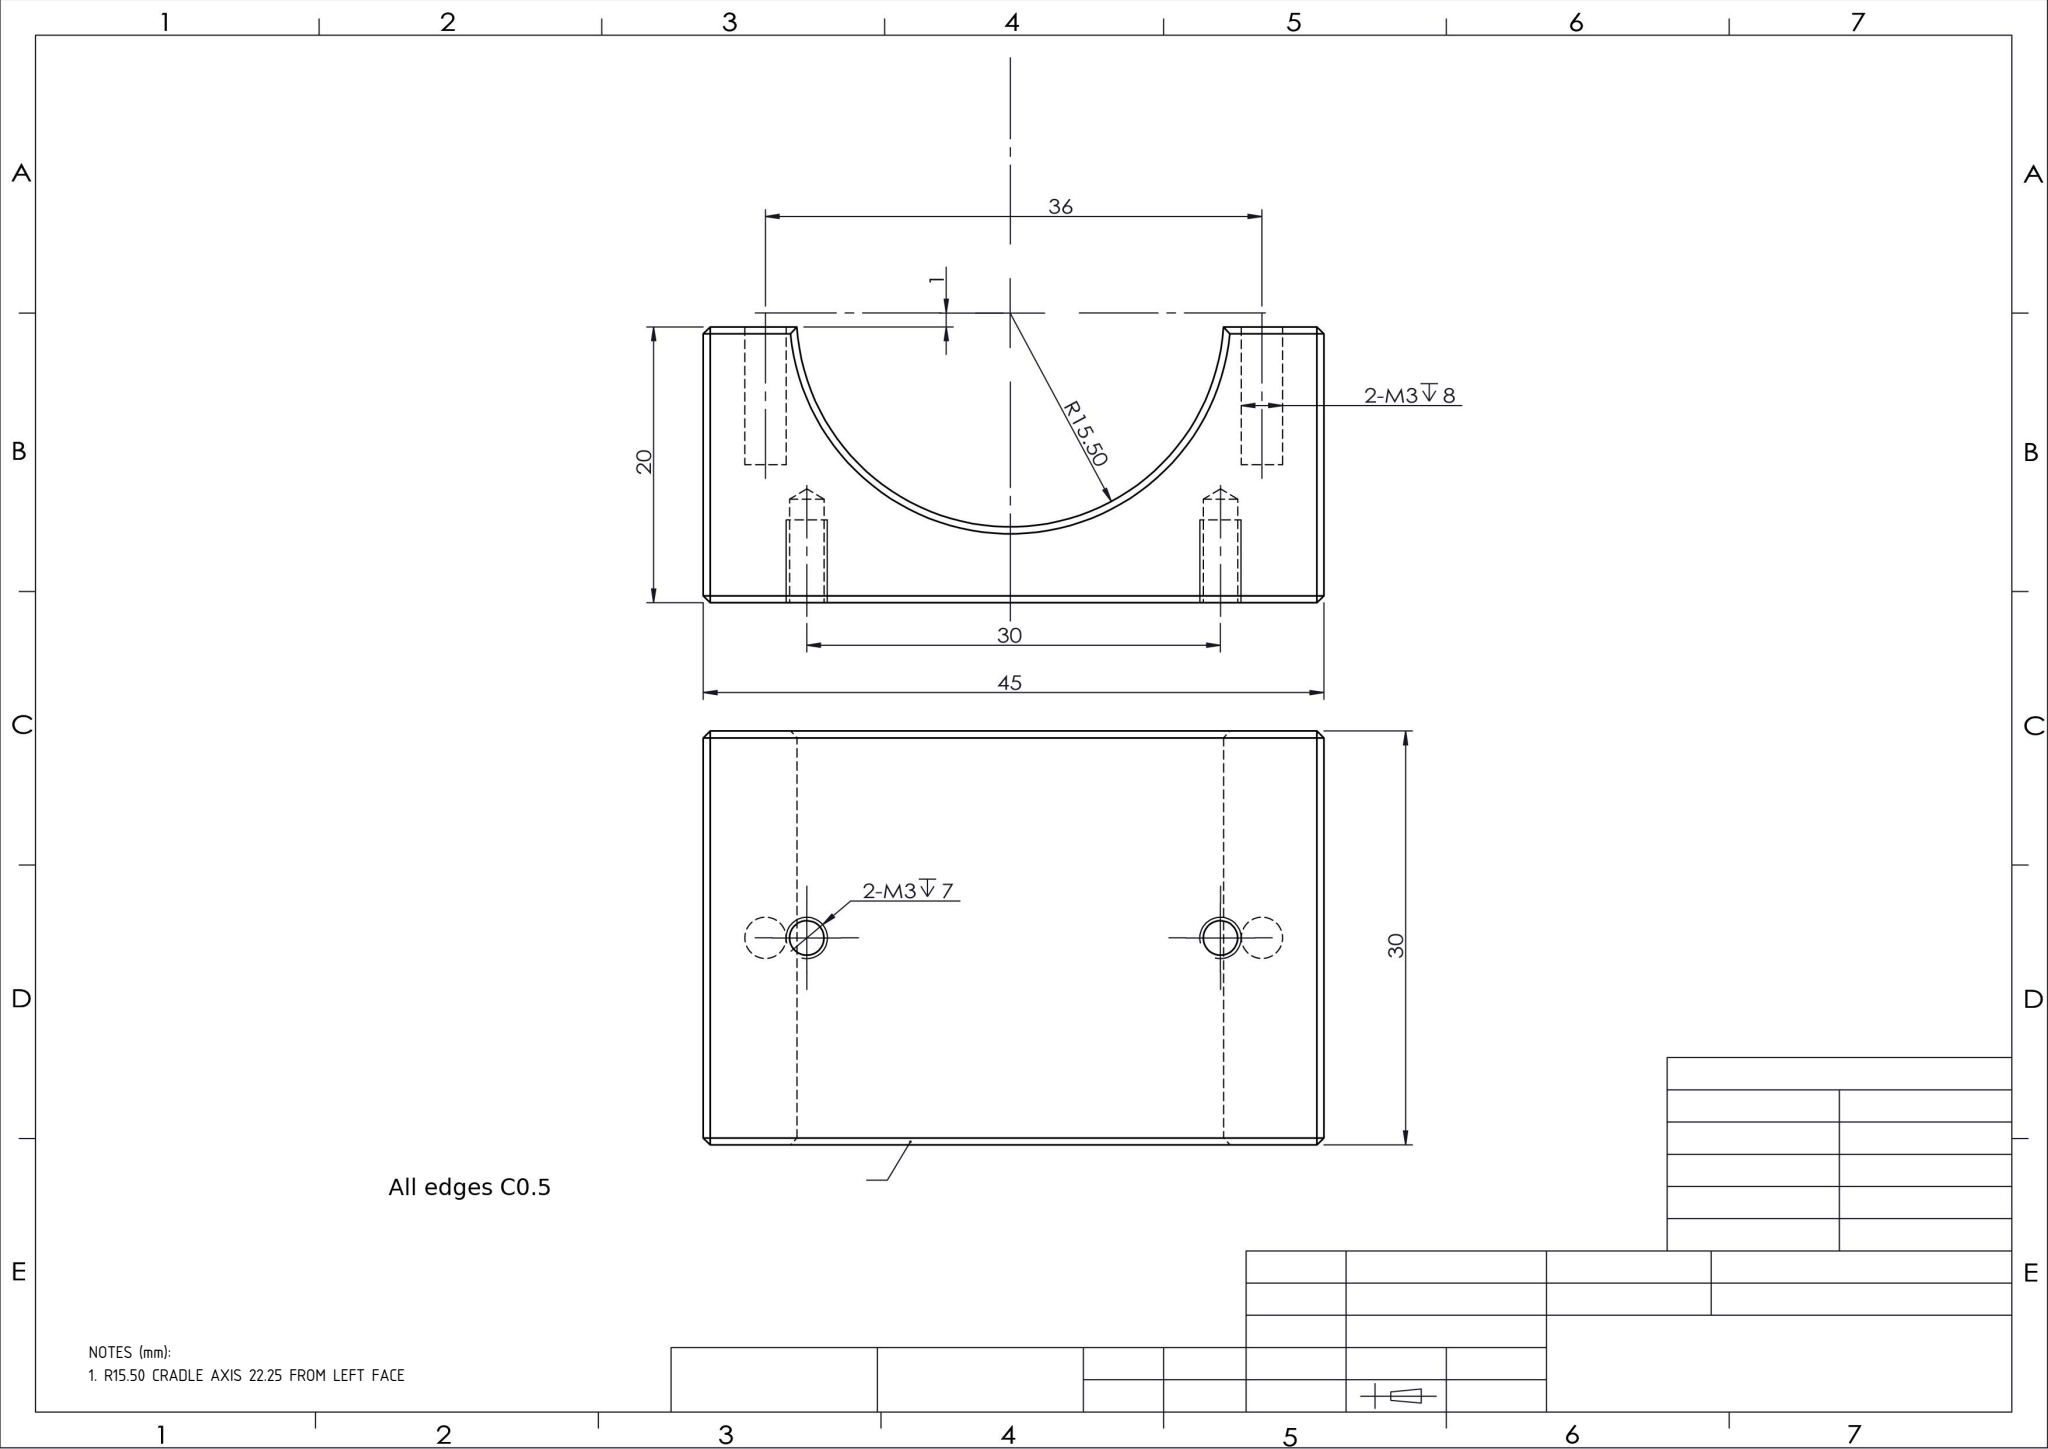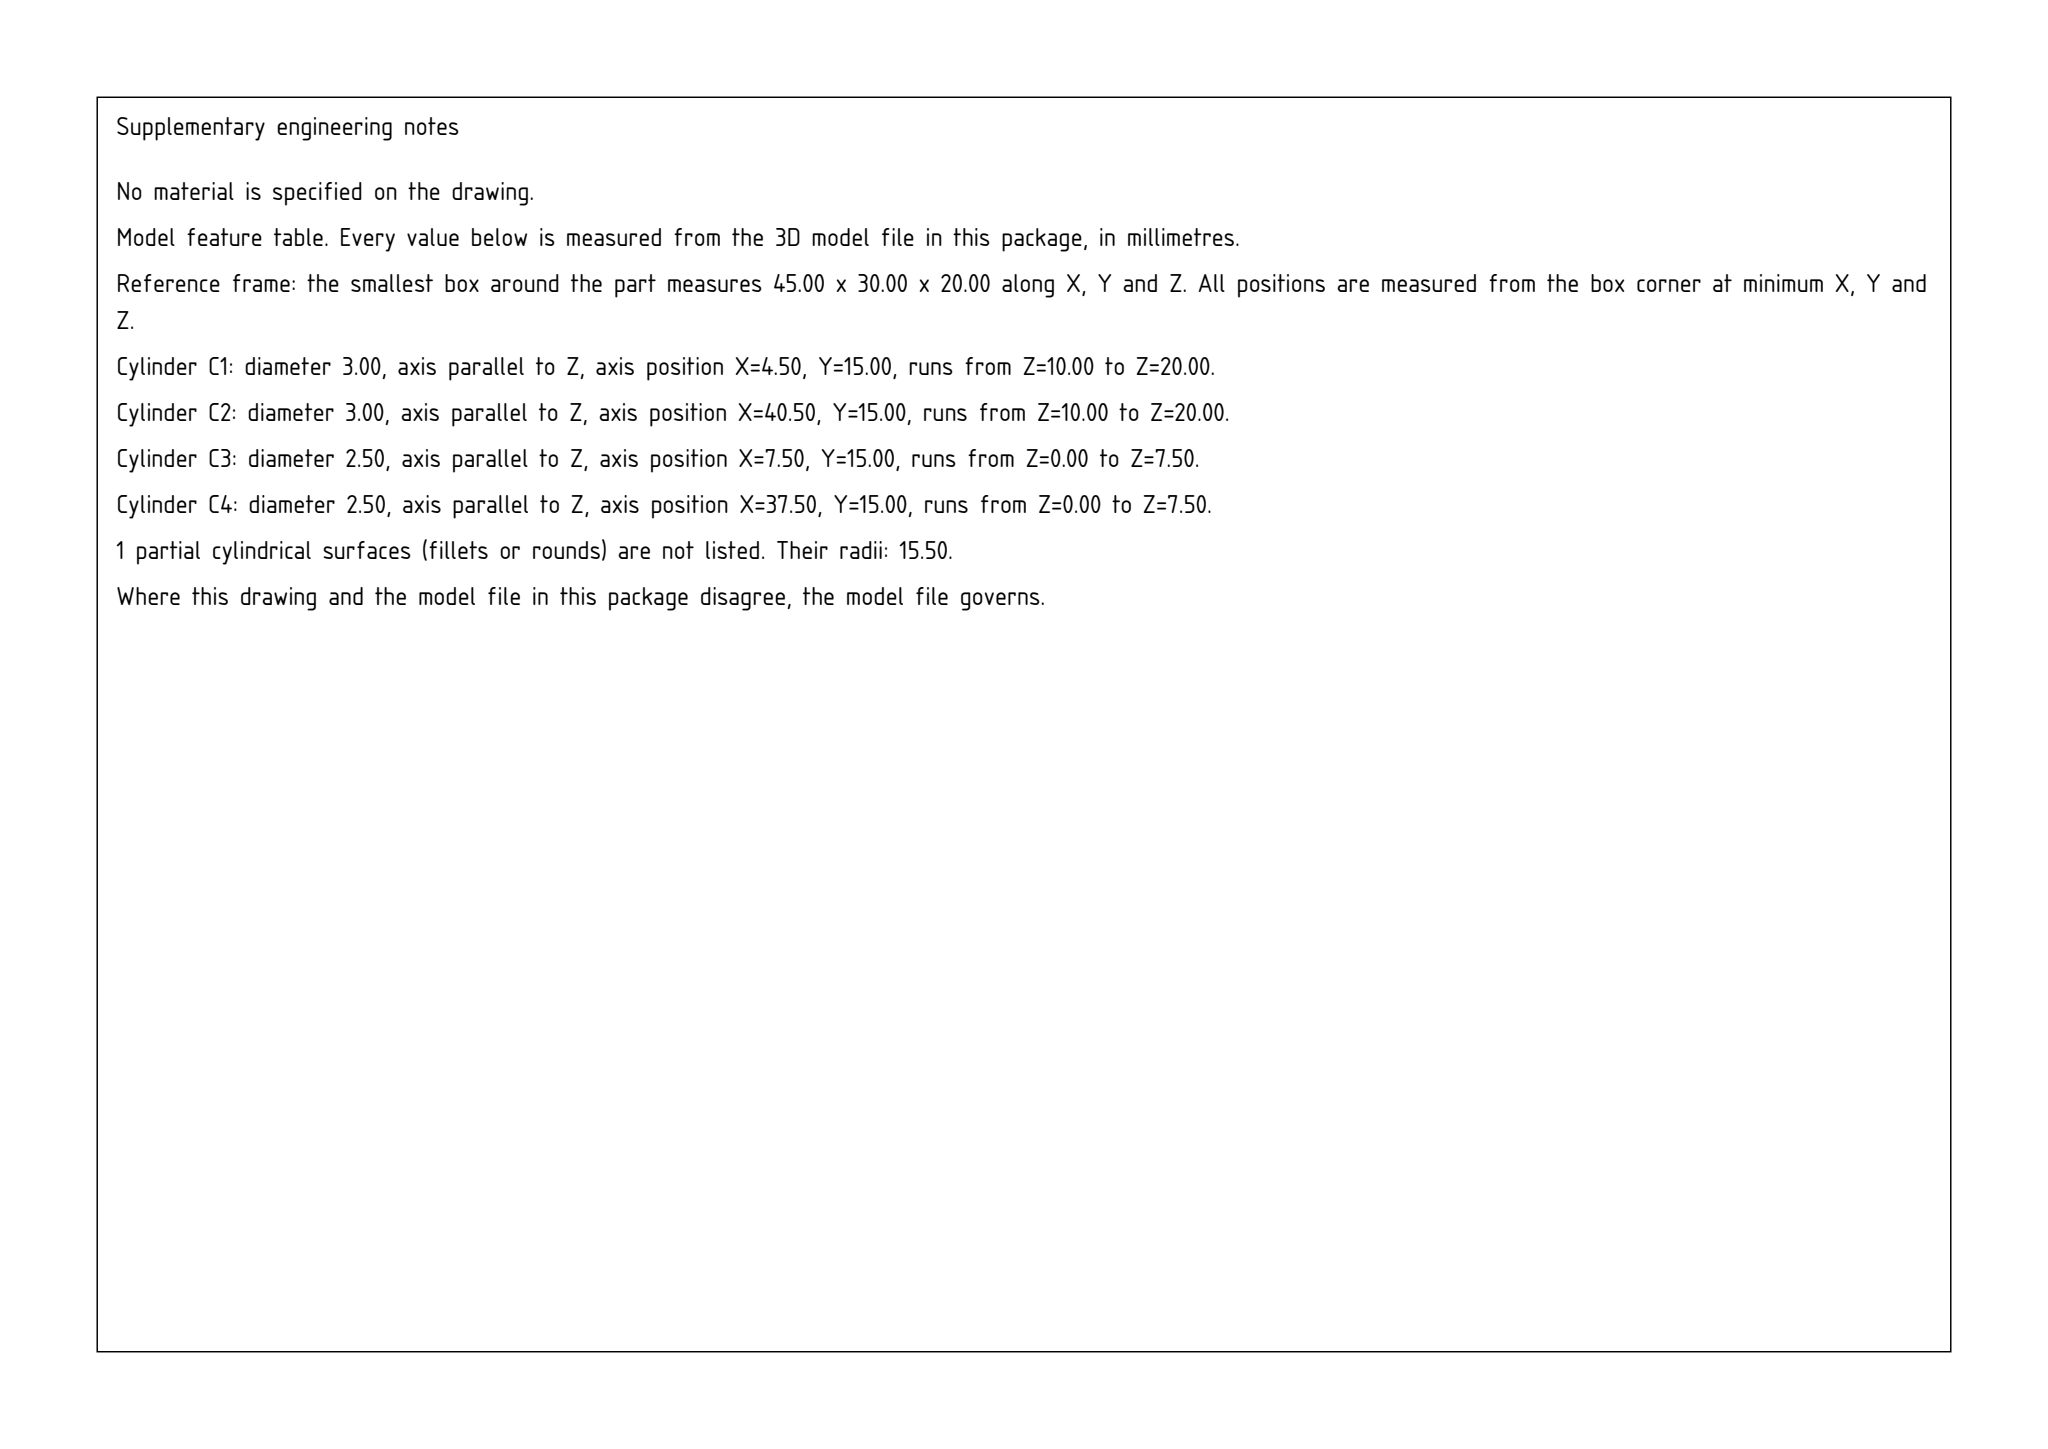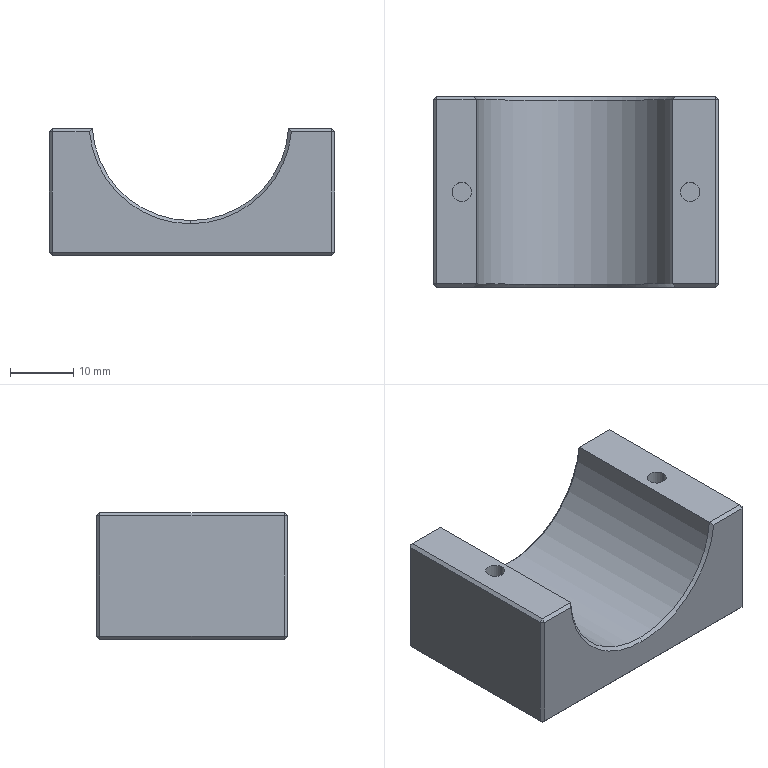Part | SolidWorks | mm | 1 solid | 47 faces | box 45 x 30 x 20 mm | volume 16340 mm3 | plane 31 | cylinder 9 | cone 7 | commonest cylinder face diameters 2.5 x4 3 x4 31 x1
Drawing notes:
R15.50 CRADLE AXIS 22.25 FROM LEFT FACE | from the solid: cylinder dia 31.0 axis y at x=22.25 (bbox x 0-45)
build123d program:
from build123d import *

# Parameters (mm, degrees)
SKETCH1_W             = 45
SKETCH1_H             = 30
BOSS_EXTRUDE1_DEPTH   = 20
SKETCH2_R             = 15.5
CUT_EXTRUDE1_DEPTH    = 58.663
SKETCH3_R             = 1.5
CUT_EXTRUDE2_DEPTH    = 10
M3_TAPPED_HOLE1_D     = 2.5
M3_TAPPED_HOLE1_DEPTH = 7.5
M3_TAPPED_HOLE1_TIP   = 0.7511
CHAMFER1_SIZE         = 0.5


with BuildPart() as part:
    # Sketch1 → Boss-Extrude1 (new body)
    with BuildSketch(Plane.XY):
        with Locations((22.5, 15)):
            Rectangle(SKETCH1_W, SKETCH1_H)
    extrude(amount=BOSS_EXTRUDE1_DEPTH)

    # Sketch2 → Cut-Extrude1 (cut, through all)
    with BuildSketch(Plane(origin=(0, 30, 0), x_dir=(1, 0, 0), z_dir=(0, 1, 0))):
        with Locations((22.254, -21)):
            Circle(SKETCH2_R)
    extrude(amount=-CUT_EXTRUDE1_DEPTH, mode=Mode.SUBTRACT)

    # Sketch3 → Cut-Extrude2 (cut)
    with BuildSketch(Plane.XY.offset(20)):
        with Locations((4.5, 15)):
            Circle(SKETCH3_R)
        with Locations((40.5, 15)):
            Circle(SKETCH3_R)
    extrude(amount=-CUT_EXTRUDE2_DEPTH, mode=Mode.SUBTRACT)

    # M3 Tapped Hole1
    with Locations(Plane(origin=(0, 0, 0), x_dir=(-1, 0, 0), z_dir=(0, 0, -1))):
        with Locations((-37.5, 15), (-7.5, 15)):
            Hole(M3_TAPPED_HOLE1_D / 2, depth=M3_TAPPED_HOLE1_DEPTH)
            with Locations((0, 0, -(M3_TAPPED_HOLE1_DEPTH + M3_TAPPED_HOLE1_TIP / 2))):  # 118° drill point
                Cone(0, M3_TAPPED_HOLE1_D / 2, M3_TAPPED_HOLE1_TIP, mode=Mode.SUBTRACT)

    # Chamfer1
    chamfer1_edges = [part.edges().sort_by_distance(p)[0] for p in [
        (45, 15, 20),
        (41.361, 30, 20),
        (41.361, 0, 20),
        (3.393, 30, 20),
        (22.254, 0, 5.5),
        (22.254, 30, 5.5),
        (0, 15, 20),
        (22.5, 30, 0),
        (45, 15, 0),
        (22.5, 0, 0),
        (0, 15, 0),
        (3.393, 0, 20),
        (0, 30, 10),
        (45, 30, 10),
        (45, 0, 10),
        (0, 0, 10),
    ]]
    chamfer(chamfer1_edges, length=CHAMFER1_SIZE)


solid = part.part